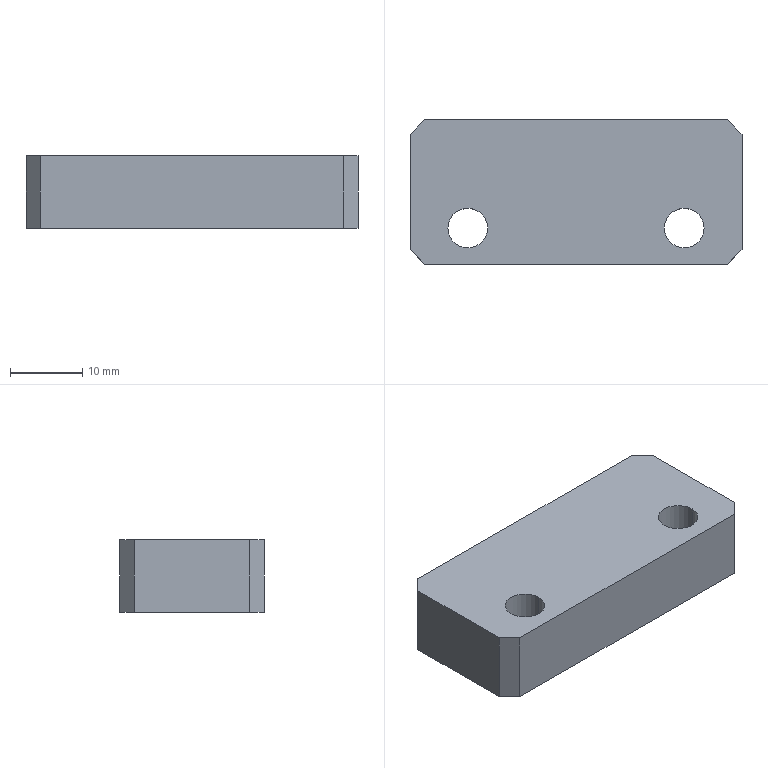Component | SolidWorks | P-SLJ-002-2_SL-26-1 | 1 solid | 14 faces | box 46 x 20 x 10 mm | volume 8645 mm3 | plane 10 | cylinder 4 | commonest cylinder face diameters 5.5 x4
build123d program:
from build123d import *

# Parameters (mm, degrees)
SKETCH1_W            = 46
SKETCH1_H            = 20
BOSS_EXTRUDE1_DEPTH  = 10
M5_CLEARANCE_HOLE1_D = 5.5
CHAMFER1_SIZE        = 2


with BuildPart() as part:
    # Sketch1 → Boss-Extrude1 (new body)
    with BuildSketch(Plane.XY):
        with Locations((23, 10)):
            Rectangle(SKETCH1_W, SKETCH1_H)
    extrude(amount=BOSS_EXTRUDE1_DEPTH)

    # M5 Clearance Hole1 (through all)
    with Locations(Plane.XY.offset(10)):
        with Locations((8, 5), (38, 5)):
            Hole(M5_CLEARANCE_HOLE1_D / 2)

    # Chamfer1
    chamfer1_edges = [part.edges().sort_by_distance(p)[0] for p in [
        (0, 20, 5),
        (46, 20, 5),
        (46, 0, 5),
        (0, 0, 5),
    ]]
    chamfer(chamfer1_edges, length=CHAMFER1_SIZE)


solid = part.part

# Placed as in the assembly
solid = solid.moved(Location((-216, -83, 796.634), (0, 0, 0)))
STEP:
#1=CARTESIAN_POINT('',(-6.9,-3.071,31.757));
#2=VERTEX_POINT('',#1);
#3=CARTESIAN_POINT('',(-7.116,-3.071,31.757));
#4=VERTEX_POINT('',#3);
#5=CARTESIAN_POINT('',(-7.008,-3.071,31.757));
#6=DIRECTION('',(0.,0.,-1.));
#7=DIRECTION('',(-1.,0.,0.));
#8=AXIS2_PLACEMENT_3D('',#5,#6,#7);
#9=CIRCLE('',#8,0.1083);
#10=EDGE_CURVE('',#2,#4,#9,.T.);
#11=ORIENTED_EDGE('',*,*,#10,.F.);
#12=CARTESIAN_POINT('',(-6.9,-3.071,31.364));
#13=VERTEX_POINT('',#12);
#14=CARTESIAN_POINT('',(-6.9,-3.071,31.364));
#15=DIRECTION('',(0.,0.,-1.));
#16=VECTOR('',#15,39.37);
#17=LINE('',#14,#16);
#18=EDGE_CURVE('',#2,#13,#17,.T.);
#19=ORIENTED_EDGE('',*,*,#18,.T.);
#20=CARTESIAN_POINT('',(-7.116,-3.071,31.364));
#21=VERTEX_POINT('',#20);
#22=CARTESIAN_POINT('',(-7.008,-3.071,31.364));
#23=DIRECTION('',(0.,0.,-1.));
#24=DIRECTION('',(-1.,0.,0.));
#25=AXIS2_PLACEMENT_3D('',#22,#23,#24);
#26=CIRCLE('',#25,0.1083);
#27=EDGE_CURVE('',#13,#21,#26,.T.);
#28=ORIENTED_EDGE('',*,*,#27,.T.);
#29=CARTESIAN_POINT('',(-7.116,-3.071,31.364));
#30=DIRECTION('',(0.,0.,-1.));
#31=VECTOR('',#30,39.37);
#32=LINE('',#29,#31);
#33=EDGE_CURVE('',#4,#21,#32,.T.);
#34=ORIENTED_EDGE('',*,*,#33,.F.);
#35=EDGE_LOOP('',(#11,#19,#28,#34));
#36=FACE_OUTER_BOUND('',#35,.T.);
#37=CARTESIAN_POINT('',(-7.008,-3.071,31.364));
#38=DIRECTION('',(0.,0.,-1.));
#39=DIRECTION('',(-1.,0.,0.));
#40=AXIS2_PLACEMENT_3D('',#37,#38,#39);
#41=CYLINDRICAL_SURFACE('',#40,0.1083);
#42=ADVANCED_FACE('',(#36),#41,.F.);
#43=CARTESIAN_POINT('',(-8.081,-3.071,31.757));
#44=VERTEX_POINT('',#43);
#45=CARTESIAN_POINT('',(-8.297,-3.071,31.757));
#46=VERTEX_POINT('',#45);
#47=CARTESIAN_POINT('',(-8.189,-3.071,31.757));
#48=DIRECTION('',(0.,0.,-1.));
#49=DIRECTION('',(-1.,0.,0.));
#50=AXIS2_PLACEMENT_3D('',#47,#48,#49);
#51=CIRCLE('',#50,0.1083);
#52=EDGE_CURVE('',#44,#46,#51,.T.);
#53=ORIENTED_EDGE('',*,*,#52,.F.);
#54=CARTESIAN_POINT('',(-8.081,-3.071,31.364));
#55=VERTEX_POINT('',#54);
#56=CARTESIAN_POINT('',(-8.081,-3.071,31.364));
#57=DIRECTION('',(0.,0.,-1.));
#58=VECTOR('',#57,39.37);
#59=LINE('',#56,#58);
#60=EDGE_CURVE('',#44,#55,#59,.T.);
#61=ORIENTED_EDGE('',*,*,#60,.T.);
#62=CARTESIAN_POINT('',(-8.297,-3.071,31.364));
#63=VERTEX_POINT('',#62);
#64=CARTESIAN_POINT('',(-8.189,-3.071,31.364));
#65=DIRECTION('',(0.,0.,-1.));
#66=DIRECTION('',(-1.,0.,0.));
#67=AXIS2_PLACEMENT_3D('',#64,#65,#66);
#68=CIRCLE('',#67,0.1083);
#69=EDGE_CURVE('',#55,#63,#68,.T.);
#70=ORIENTED_EDGE('',*,*,#69,.T.);
#71=CARTESIAN_POINT('',(-8.297,-3.071,31.364));
#72=DIRECTION('',(0.,0.,-1.));
#73=VECTOR('',#72,39.37);
#74=LINE('',#71,#73);
#75=EDGE_CURVE('',#46,#63,#74,.T.);
#76=ORIENTED_EDGE('',*,*,#75,.F.);
#77=EDGE_LOOP('',(#53,#61,#70,#76));
#78=FACE_OUTER_BOUND('',#77,.T.);
#79=CARTESIAN_POINT('',(-8.189,-3.071,31.364));
#80=DIRECTION('',(0.,0.,-1.));
#81=DIRECTION('',(-1.,0.,0.));
#82=AXIS2_PLACEMENT_3D('',#79,#80,#81);
#83=CYLINDRICAL_SURFACE('',#82,0.1083);
#84=ADVANCED_FACE('',(#78),#83,.F.);
#85=CARTESIAN_POINT('',(-6.693,-2.559,31.757));
#86=VERTEX_POINT('',#85);
#87=CARTESIAN_POINT('',(-6.693,-3.189,31.757));
#88=VERTEX_POINT('',#87);
#89=CARTESIAN_POINT('',(-6.693,-3.268,31.757));
#90=DIRECTION('',(-0.,-1.,0.));
#91=VECTOR('',#90,39.37);
#92=LINE('',#89,#91);
#93=EDGE_CURVE('',#86,#88,#92,.T.);
#94=ORIENTED_EDGE('',*,*,#93,.T.);
#95=CARTESIAN_POINT('',(-6.693,-3.189,31.364));
#96=VERTEX_POINT('',#95);
#97=CARTESIAN_POINT('',(-6.693,-3.189,31.364));
#98=DIRECTION('',(0.,0.,-1.));
#99=VECTOR('',#98,39.37);
#100=LINE('',#97,#99);
#101=EDGE_CURVE('',#88,#96,#100,.T.);
#102=ORIENTED_EDGE('',*,*,#101,.T.);
#103=CARTESIAN_POINT('',(-6.693,-2.559,31.364));
#104=VERTEX_POINT('',#103);
#105=CARTESIAN_POINT('',(-6.693,-3.268,31.364));
#106=DIRECTION('',(-0.,-1.,0.));
#107=VECTOR('',#106,39.37);
#108=LINE('',#105,#107);
#109=EDGE_CURVE('',#104,#96,#108,.T.);
#110=ORIENTED_EDGE('',*,*,#109,.F.);
#111=CARTESIAN_POINT('',(-6.693,-2.559,31.364));
#112=DIRECTION('',(0.,0.,1.));
#113=VECTOR('',#112,39.37);
#114=LINE('',#111,#113);
#115=EDGE_CURVE('',#104,#86,#114,.T.);
#116=ORIENTED_EDGE('',*,*,#115,.T.);
#117=EDGE_LOOP('',(#94,#102,#110,#116));
#118=FACE_OUTER_BOUND('',#117,.T.);
#119=CARTESIAN_POINT('',(-6.693,-3.268,31.364));
#120=DIRECTION('',(-1.,0.,0.));
#121=DIRECTION('',(0.,0.,1.));
#122=AXIS2_PLACEMENT_3D('',#119,#120,#121);
#123=PLANE('',#122);
#124=ADVANCED_FACE('',(#118),#123,.F.);
#125=CARTESIAN_POINT('',(-6.772,-3.268,31.757));
#126=VERTEX_POINT('',#125);
#127=CARTESIAN_POINT('',(-8.425,-3.268,31.757));
#128=VERTEX_POINT('',#127);
#129=CARTESIAN_POINT('',(-6.693,-3.268,31.757));
#130=DIRECTION('',(-1.,0.,0.));
#131=VECTOR('',#130,39.37);
#132=LINE('',#129,#131);
#133=EDGE_CURVE('',#126,#128,#132,.T.);
#134=ORIENTED_EDGE('',*,*,#133,.T.);
#135=CARTESIAN_POINT('',(-8.425,-3.268,31.364));
#136=VERTEX_POINT('',#135);
#137=CARTESIAN_POINT('',(-8.425,-3.268,31.364));
#138=DIRECTION('',(0.,0.,-1.));
#139=VECTOR('',#138,39.37);
#140=LINE('',#137,#139);
#141=EDGE_CURVE('',#128,#136,#140,.T.);
#142=ORIENTED_EDGE('',*,*,#141,.T.);
#143=CARTESIAN_POINT('',(-6.772,-3.268,31.364));
#144=VERTEX_POINT('',#143);
#145=CARTESIAN_POINT('',(-6.693,-3.268,31.364));
#146=DIRECTION('',(-1.,0.,0.));
#147=VECTOR('',#146,39.37);
#148=LINE('',#145,#147);
#149=EDGE_CURVE('',#144,#136,#148,.T.);
#150=ORIENTED_EDGE('',*,*,#149,.F.);
#151=CARTESIAN_POINT('',(-6.772,-3.268,31.364));
#152=DIRECTION('',(0.,0.,1.));
#153=VECTOR('',#152,39.37);
#154=LINE('',#151,#153);
#155=EDGE_CURVE('',#144,#126,#154,.T.);
#156=ORIENTED_EDGE('',*,*,#155,.T.);
#157=EDGE_LOOP('',(#134,#142,#150,#156));
#158=FACE_OUTER_BOUND('',#157,.T.);
#159=CARTESIAN_POINT('',(-6.693,-3.268,31.364));
#160=DIRECTION('',(0.,1.,0.));
#161=DIRECTION('',(0.,0.,-1.));
#162=AXIS2_PLACEMENT_3D('',#159,#160,#161);
#163=PLANE('',#162);
#164=ADVANCED_FACE('',(#158),#163,.F.);
#165=CARTESIAN_POINT('',(-8.504,-3.189,31.364));
#166=VERTEX_POINT('',#165);
#167=CARTESIAN_POINT('',(-8.504,-2.559,31.364));
#168=VERTEX_POINT('',#167);
#169=CARTESIAN_POINT('',(-8.504,-3.268,31.364));
#170=DIRECTION('',(0.,1.,0.));
#171=VECTOR('',#170,39.37);
#172=LINE('',#169,#171);
#173=EDGE_CURVE('',#166,#168,#172,.T.);
#174=ORIENTED_EDGE('',*,*,#173,.F.);
#175=CARTESIAN_POINT('',(-8.504,-3.189,31.757));
#176=VERTEX_POINT('',#175);
#177=CARTESIAN_POINT('',(-8.504,-3.189,31.364));
#178=DIRECTION('',(0.,0.,1.));
#179=VECTOR('',#178,39.37);
#180=LINE('',#177,#179);
#181=EDGE_CURVE('',#166,#176,#180,.T.);
#182=ORIENTED_EDGE('',*,*,#181,.T.);
#183=CARTESIAN_POINT('',(-8.504,-2.559,31.757));
#184=VERTEX_POINT('',#183);
#185=CARTESIAN_POINT('',(-8.504,-3.268,31.757));
#186=DIRECTION('',(0.,1.,0.));
#187=VECTOR('',#186,39.37);
#188=LINE('',#185,#187);
#189=EDGE_CURVE('',#176,#184,#188,.T.);
#190=ORIENTED_EDGE('',*,*,#189,.T.);
#191=CARTESIAN_POINT('',(-8.504,-2.559,31.364));
#192=DIRECTION('',(0.,0.,-1.));
#193=VECTOR('',#192,39.37);
#194=LINE('',#191,#193);
#195=EDGE_CURVE('',#184,#168,#194,.T.);
#196=ORIENTED_EDGE('',*,*,#195,.T.);
#197=EDGE_LOOP('',(#174,#182,#190,#196));
#198=FACE_OUTER_BOUND('',#197,.T.);
#199=CARTESIAN_POINT('',(-8.504,-3.268,31.364));
#200=DIRECTION('',(1.,-0.,0.));
#201=DIRECTION('',(0.,0.,-1.));
#202=AXIS2_PLACEMENT_3D('',#199,#200,#201);
#203=PLANE('',#202);
#204=ADVANCED_FACE('',(#198),#203,.F.);
#205=CARTESIAN_POINT('',(-8.425,-2.48,31.364));
#206=VERTEX_POINT('',#205);
#207=CARTESIAN_POINT('',(-6.772,-2.48,31.364));
#208=VERTEX_POINT('',#207);
#209=CARTESIAN_POINT('',(-6.693,-2.48,31.364));
#210=DIRECTION('',(1.,-0.,0.));
#211=VECTOR('',#210,39.37);
#212=LINE('',#209,#211);
#213=EDGE_CURVE('',#206,#208,#212,.T.);
#214=ORIENTED_EDGE('',*,*,#213,.F.);
#215=CARTESIAN_POINT('',(-8.425,-2.48,31.757));
#216=VERTEX_POINT('',#215);
#217=CARTESIAN_POINT('',(-8.425,-2.48,31.364));
#218=DIRECTION('',(0.,0.,1.));
#219=VECTOR('',#218,39.37);
#220=LINE('',#217,#219);
#221=EDGE_CURVE('',#206,#216,#220,.T.);
#222=ORIENTED_EDGE('',*,*,#221,.T.);
#223=CARTESIAN_POINT('',(-6.772,-2.48,31.757));
#224=VERTEX_POINT('',#223);
#225=CARTESIAN_POINT('',(-6.693,-2.48,31.757));
#226=DIRECTION('',(1.,-0.,0.));
#227=VECTOR('',#226,39.37);
#228=LINE('',#225,#227);
#229=EDGE_CURVE('',#216,#224,#228,.T.);
#230=ORIENTED_EDGE('',*,*,#229,.T.);
#231=CARTESIAN_POINT('',(-6.772,-2.48,31.364));
#232=DIRECTION('',(0.,0.,-1.));
#233=VECTOR('',#232,39.37);
#234=LINE('',#231,#233);
#235=EDGE_CURVE('',#224,#208,#234,.T.);
#236=ORIENTED_EDGE('',*,*,#235,.T.);
#237=EDGE_LOOP('',(#214,#222,#230,#236));
#238=FACE_OUTER_BOUND('',#237,.T.);
#239=CARTESIAN_POINT('',(-6.693,-2.48,31.364));
#240=DIRECTION('',(-0.,-1.,0.));
#241=DIRECTION('',(0.,0.,1.));
#242=AXIS2_PLACEMENT_3D('',#239,#240,#241);
#243=PLANE('',#242);
#244=ADVANCED_FACE('',(#238),#243,.F.);
#245=CARTESIAN_POINT('',(-7.008,-3.071,31.364));
#246=DIRECTION('',(0.,0.,-1.));
#247=DIRECTION('',(-1.,0.,0.));
#248=AXIS2_PLACEMENT_3D('',#245,#246,#247);
#249=CIRCLE('',#248,0.1083);
#250=EDGE_CURVE('',#21,#13,#249,.T.);
#251=ORIENTED_EDGE('',*,*,#250,.F.);
#252=ORIENTED_EDGE('',*,*,#27,.F.);
#253=EDGE_LOOP('',(#251,#252));
#254=FACE_BOUND('',#253,.T.);
#255=CARTESIAN_POINT('',(-8.189,-3.071,31.364));
#256=DIRECTION('',(0.,0.,-1.));
#257=DIRECTION('',(-1.,0.,0.));
#258=AXIS2_PLACEMENT_3D('',#255,#256,#257);
#259=CIRCLE('',#258,0.1083);
#260=EDGE_CURVE('',#63,#55,#259,.T.);
#261=ORIENTED_EDGE('',*,*,#260,.F.);
#262=ORIENTED_EDGE('',*,*,#69,.F.);
#263=EDGE_LOOP('',(#261,#262));
#264=FACE_BOUND('',#263,.T.);
#265=ORIENTED_EDGE('',*,*,#149,.T.);
#266=CARTESIAN_POINT('',(-8.504,-3.189,31.364));
#267=DIRECTION('',(-0.7071,0.7071,0.));
#268=VECTOR('',#267,39.37);
#269=LINE('',#266,#268);
#270=EDGE_CURVE('',#136,#166,#269,.T.);
#271=ORIENTED_EDGE('',*,*,#270,.T.);
#272=ORIENTED_EDGE('',*,*,#173,.T.);
#273=CARTESIAN_POINT('',(-8.425,-2.48,31.364));
#274=DIRECTION('',(0.7071,0.7071,0.));
#275=VECTOR('',#274,39.37);
#276=LINE('',#273,#275);
#277=EDGE_CURVE('',#168,#206,#276,.T.);
#278=ORIENTED_EDGE('',*,*,#277,.T.);
#279=ORIENTED_EDGE('',*,*,#213,.T.);
#280=CARTESIAN_POINT('',(-6.693,-2.559,31.364));
#281=DIRECTION('',(0.7071,-0.7071,0.));
#282=VECTOR('',#281,39.37);
#283=LINE('',#280,#282);
#284=EDGE_CURVE('',#208,#104,#283,.T.);
#285=ORIENTED_EDGE('',*,*,#284,.T.);
#286=ORIENTED_EDGE('',*,*,#109,.T.);
#287=CARTESIAN_POINT('',(-6.772,-3.268,31.364));
#288=DIRECTION('',(-0.7071,-0.7071,0.));
#289=VECTOR('',#288,39.37);
#290=LINE('',#287,#289);
#291=EDGE_CURVE('',#96,#144,#290,.T.);
#292=ORIENTED_EDGE('',*,*,#291,.T.);
#293=EDGE_LOOP('',(#265,#271,#272,#278,#279,#285,#286,#292));
#294=FACE_OUTER_BOUND('',#293,.T.);
#295=CARTESIAN_POINT('',(-6.693,-3.268,31.364));
#296=DIRECTION('',(0.,0.,1.));
#297=DIRECTION('',(1.,-0.,0.));
#298=AXIS2_PLACEMENT_3D('',#295,#296,#297);
#299=PLANE('',#298);
#300=ADVANCED_FACE('',(#254,#264,#294),#299,.F.);
#301=CARTESIAN_POINT('',(-7.008,-3.071,31.757));
#302=DIRECTION('',(0.,0.,-1.));
#303=DIRECTION('',(-1.,0.,0.));
#304=AXIS2_PLACEMENT_3D('',#301,#302,#303);
#305=CIRCLE('',#304,0.1083);
#306=EDGE_CURVE('',#4,#2,#305,.T.);
#307=ORIENTED_EDGE('',*,*,#306,.T.);
#308=ORIENTED_EDGE('',*,*,#10,.T.);
#309=EDGE_LOOP('',(#307,#308));
#310=FACE_BOUND('',#309,.T.);
#311=CARTESIAN_POINT('',(-8.189,-3.071,31.757));
#312=DIRECTION('',(0.,0.,-1.));
#313=DIRECTION('',(-1.,0.,0.));
#314=AXIS2_PLACEMENT_3D('',#311,#312,#313);
#315=CIRCLE('',#314,0.1083);
#316=EDGE_CURVE('',#46,#44,#315,.T.);
#317=ORIENTED_EDGE('',*,*,#316,.T.);
#318=ORIENTED_EDGE('',*,*,#52,.T.);
#319=EDGE_LOOP('',(#317,#318));
#320=FACE_BOUND('',#319,.T.);
#321=ORIENTED_EDGE('',*,*,#189,.F.);
#322=CARTESIAN_POINT('',(-7.559,-4.134,31.757));
#323=DIRECTION('',(0.7071,-0.7071,0.));
#324=VECTOR('',#323,39.37);
#325=LINE('',#322,#324);
#326=EDGE_CURVE('',#176,#128,#325,.T.);
#327=ORIENTED_EDGE('',*,*,#326,.T.);
#328=ORIENTED_EDGE('',*,*,#133,.F.);
#329=CARTESIAN_POINT('',(-6.732,-3.228,31.757));
#330=DIRECTION('',(0.7071,0.7071,0.));
#331=VECTOR('',#330,39.37);
#332=LINE('',#329,#331);
#333=EDGE_CURVE('',#126,#88,#332,.T.);
#334=ORIENTED_EDGE('',*,*,#333,.T.);
#335=ORIENTED_EDGE('',*,*,#93,.F.);
#336=CARTESIAN_POINT('',(-6.339,-2.913,31.757));
#337=DIRECTION('',(-0.7071,0.7071,0.));
#338=VECTOR('',#337,39.37);
#339=LINE('',#336,#338);
#340=EDGE_CURVE('',#86,#224,#339,.T.);
#341=ORIENTED_EDGE('',*,*,#340,.T.);
#342=ORIENTED_EDGE('',*,*,#229,.F.);
#343=CARTESIAN_POINT('',(-7.953,-2.008,31.757));
#344=DIRECTION('',(-0.7071,-0.7071,0.));
#345=VECTOR('',#344,39.37);
#346=LINE('',#343,#345);
#347=EDGE_CURVE('',#216,#184,#346,.T.);
#348=ORIENTED_EDGE('',*,*,#347,.T.);
#349=EDGE_LOOP('',(#321,#327,#328,#334,#335,#341,#342,#348));
#350=FACE_OUTER_BOUND('',#349,.T.);
#351=CARTESIAN_POINT('',(-6.693,-3.268,31.757));
#352=DIRECTION('',(0.,0.,1.));
#353=DIRECTION('',(1.,-0.,0.));
#354=AXIS2_PLACEMENT_3D('',#351,#352,#353);
#355=PLANE('',#354);
#356=ADVANCED_FACE('',(#310,#320,#350),#355,.T.);
#357=ORIENTED_EDGE('',*,*,#60,.F.);
#358=ORIENTED_EDGE('',*,*,#316,.F.);
#359=ORIENTED_EDGE('',*,*,#75,.T.);
#360=ORIENTED_EDGE('',*,*,#260,.T.);
#361=EDGE_LOOP('',(#357,#358,#359,#360));
#362=FACE_OUTER_BOUND('',#361,.T.);
#363=CARTESIAN_POINT('',(-8.189,-3.071,31.364));
#364=DIRECTION('',(0.,0.,-1.));
#365=DIRECTION('',(-1.,0.,0.));
#366=AXIS2_PLACEMENT_3D('',#363,#364,#365);
#367=CYLINDRICAL_SURFACE('',#366,0.1083);
#368=ADVANCED_FACE('',(#362),#367,.F.);
#369=ORIENTED_EDGE('',*,*,#18,.F.);
#370=ORIENTED_EDGE('',*,*,#306,.F.);
#371=ORIENTED_EDGE('',*,*,#33,.T.);
#372=ORIENTED_EDGE('',*,*,#250,.T.);
#373=EDGE_LOOP('',(#369,#370,#371,#372));
#374=FACE_OUTER_BOUND('',#373,.T.);
#375=CARTESIAN_POINT('',(-7.008,-3.071,31.364));
#376=DIRECTION('',(0.,0.,-1.));
#377=DIRECTION('',(-1.,0.,0.));
#378=AXIS2_PLACEMENT_3D('',#375,#376,#377);
#379=CYLINDRICAL_SURFACE('',#378,0.1083);
#380=ADVANCED_FACE('',(#374),#379,.F.);
#381=ORIENTED_EDGE('',*,*,#270,.F.);
#382=ORIENTED_EDGE('',*,*,#141,.F.);
#383=ORIENTED_EDGE('',*,*,#326,.F.);
#384=ORIENTED_EDGE('',*,*,#181,.F.);
#385=EDGE_LOOP('',(#381,#382,#383,#384));
#386=FACE_OUTER_BOUND('',#385,.T.);
#387=CARTESIAN_POINT('',(-8.504,-3.189,31.364));
#388=DIRECTION('',(0.7071,0.7071,0.));
#389=DIRECTION('',(0.,0.,1.));
#390=AXIS2_PLACEMENT_3D('',#387,#388,#389);
#391=PLANE('',#390);
#392=ADVANCED_FACE('',(#386),#391,.F.);
#393=ORIENTED_EDGE('',*,*,#277,.F.);
#394=ORIENTED_EDGE('',*,*,#195,.F.);
#395=ORIENTED_EDGE('',*,*,#347,.F.);
#396=ORIENTED_EDGE('',*,*,#221,.F.);
#397=EDGE_LOOP('',(#393,#394,#395,#396));
#398=FACE_OUTER_BOUND('',#397,.T.);
#399=CARTESIAN_POINT('',(-8.425,-2.48,31.364));
#400=DIRECTION('',(0.7071,-0.7071,0.));
#401=DIRECTION('',(0.,0.,1.));
#402=AXIS2_PLACEMENT_3D('',#399,#400,#401);
#403=PLANE('',#402);
#404=ADVANCED_FACE('',(#398),#403,.F.);
#405=ORIENTED_EDGE('',*,*,#291,.F.);
#406=ORIENTED_EDGE('',*,*,#101,.F.);
#407=ORIENTED_EDGE('',*,*,#333,.F.);
#408=ORIENTED_EDGE('',*,*,#155,.F.);
#409=EDGE_LOOP('',(#405,#406,#407,#408));
#410=FACE_OUTER_BOUND('',#409,.T.);
#411=CARTESIAN_POINT('',(-6.772,-3.268,31.364));
#412=DIRECTION('',(-0.7071,0.7071,0.));
#413=DIRECTION('',(0.,0.,1.));
#414=AXIS2_PLACEMENT_3D('',#411,#412,#413);
#415=PLANE('',#414);
#416=ADVANCED_FACE('',(#410),#415,.F.);
#417=ORIENTED_EDGE('',*,*,#284,.F.);
#418=ORIENTED_EDGE('',*,*,#235,.F.);
#419=ORIENTED_EDGE('',*,*,#340,.F.);
#420=ORIENTED_EDGE('',*,*,#115,.F.);
#421=EDGE_LOOP('',(#417,#418,#419,#420));
#422=FACE_OUTER_BOUND('',#421,.T.);
#423=CARTESIAN_POINT('',(-6.693,-2.559,31.364));
#424=DIRECTION('',(-0.7071,-0.7071,0.));
#425=DIRECTION('',(0.,0.,1.));
#426=AXIS2_PLACEMENT_3D('',#423,#424,#425);
#427=PLANE('',#426);
#428=ADVANCED_FACE('',(#422),#427,.F.);
#429=CLOSED_SHELL('',(#42,#84,#124,#164,#204,#244,#300,#356,#368,#380,#392,#404,#416,#428));
#430=MANIFOLD_SOLID_BREP('',#429);
#431=CARTESIAN_POINT('',(0.,0.,0.));
#432=DIRECTION('',(0.,0.,1.));
#433=DIRECTION('',(1.,0.,0.));
#434=AXIS2_PLACEMENT_3D('',#431,#432,#433);
#435=(LENGTH_UNIT()NAMED_UNIT(*)SI_UNIT($,.METRE.));
#436=LENGTH_MEASURE_WITH_UNIT(LENGTH_MEASURE(0.0254),#435);
#437=DIMENSIONAL_EXPONENTS(1.,0.,0.,0.,0.,0.,0.);
#438=(CONVERSION_BASED_UNIT('',#436)LENGTH_UNIT()NAMED_UNIT(#437));
#439=UNCERTAINTY_MEASURE_WITH_UNIT(LENGTH_MEASURE(0.00001),#438,'','');
#440=(NAMED_UNIT(*)PLANE_ANGLE_UNIT()SI_UNIT($,.RADIAN.));
#441=(NAMED_UNIT(*)SI_UNIT($,.STERADIAN.)SOLID_ANGLE_UNIT());
#442=(GEOMETRIC_REPRESENTATION_CONTEXT(3)GLOBAL_UNCERTAINTY_ASSIGNED_CONTEXT((#439))GLOBAL_UNIT_ASSIGNED_CONTEXT((#438,#440,#441))REPRESENTATION_CONTEXT('',''));
#443=ADVANCED_BREP_SHAPE_REPRESENTATION('',(#430,#434),#442);
#444=COLOUR_RGB('',0.7922,0.8196,0.9333);
#445=FILL_AREA_STYLE_COLOUR('',#444);
#446=FILL_AREA_STYLE('',(#445));
#447=SURFACE_STYLE_FILL_AREA(#446);
#448=SURFACE_SIDE_STYLE('',(#447));
#449=SURFACE_STYLE_USAGE(.BOTH.,#448);
#450=PRESENTATION_STYLE_ASSIGNMENT((#449));
#451=STYLED_ITEM('',(#450),#430);
#452=(LENGTH_UNIT()NAMED_UNIT(*)SI_UNIT($,.METRE.));
#453=LENGTH_MEASURE_WITH_UNIT(LENGTH_MEASURE(0.0254),#452);
#454=DIMENSIONAL_EXPONENTS(1.,0.,0.,0.,0.,0.,0.);
#455=(CONVERSION_BASED_UNIT('',#453)LENGTH_UNIT()NAMED_UNIT(#454));
#456=UNCERTAINTY_MEASURE_WITH_UNIT(LENGTH_MEASURE(0.00001),#455,'','');
#457=(NAMED_UNIT(*)PLANE_ANGLE_UNIT()SI_UNIT($,.RADIAN.));
#458=(NAMED_UNIT(*)SI_UNIT($,.STERADIAN.)SOLID_ANGLE_UNIT());
#459=(GEOMETRIC_REPRESENTATION_CONTEXT(3)GLOBAL_UNCERTAINTY_ASSIGNED_CONTEXT((#456))GLOBAL_UNIT_ASSIGNED_CONTEXT((#455,#457,#458))REPRESENTATION_CONTEXT('',''));
#460=MECHANICAL_DESIGN_GEOMETRIC_PRESENTATION_REPRESENTATION('',(#451),#459);
#461=PRESENTATION_LAYER_ASSIGNMENT('','',(#451));